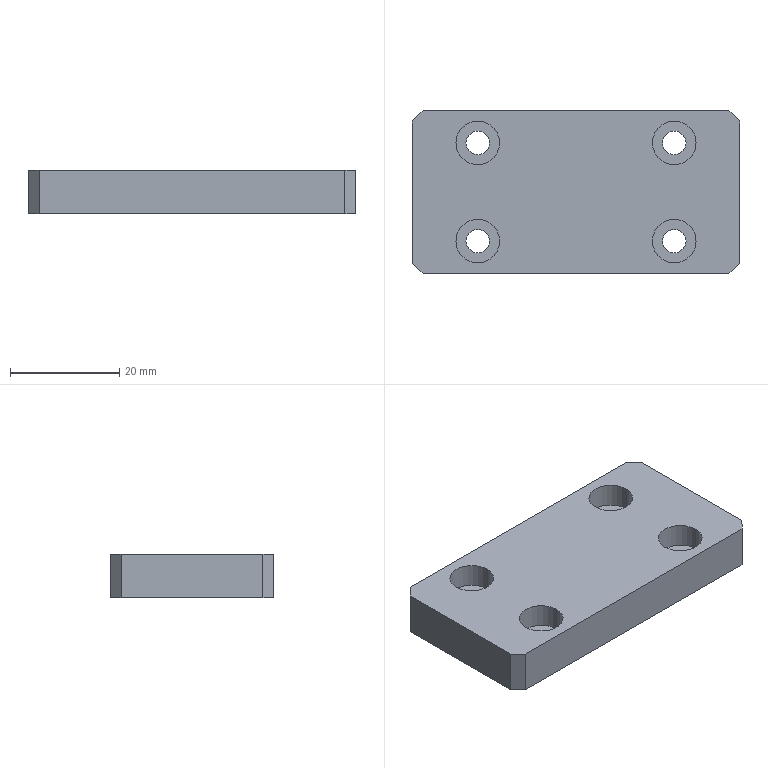Component | SolidWorks | XT-1-24-2-5 | 1 solid | 30 faces | box 60 x 30 x 8 mm | volume 13242 mm3 | cylinder 16 | plane 14 | commonest cylinder face diameters 8 x8 4.3 x8
build123d program:
from build123d import *

# Parameters (mm, degrees)
SKETCH1_W                                       = 60
SKETCH1_H                                       = 30
BOSS_EXTRUDE1_DEPTH                             = 8
M4_HEX_SOCKET_HEAD_CAP_SCREW_CBORE1_D           = 4.3
M4_HEX_SOCKET_HEAD_CAP_SCREW_CBORE1_CBORE_D     = 8
M4_HEX_SOCKET_HEAD_CAP_SCREW_CBORE1_CBORE_DEPTH = 4.4
CHAMFER1_SIZE                                   = 2


with BuildPart() as part:
    # Sketch1 → Boss-Extrude1 (new body)
    with BuildSketch(Plane.XY):
        with Locations((30, -15)):
            Rectangle(SKETCH1_W, SKETCH1_H)
    extrude(amount=BOSS_EXTRUDE1_DEPTH)

    # M4 Hex Socket Head Cap Screw CBORE1 (through all)
    with Locations(Plane.XY.offset(8)):
        with Locations((12, -6), (12, -24), (48, -6), (48, -24)):
            CounterBoreHole(M4_HEX_SOCKET_HEAD_CAP_SCREW_CBORE1_D / 2, M4_HEX_SOCKET_HEAD_CAP_SCREW_CBORE1_CBORE_D / 2, M4_HEX_SOCKET_HEAD_CAP_SCREW_CBORE1_CBORE_DEPTH)

    # Chamfer1
    chamfer1_edges = [part.edges().sort_by_distance(p)[0] for p in [
        (0, 0, 4),
        (60, 0, 4),
        (60, -30, 4),
        (0, -30, 4),
    ]]
    chamfer(chamfer1_edges, length=CHAMFER1_SIZE)


solid = part.part

# Placed as in the assembly
solid = solid.moved(Location((934.283, 92.385, -0.5), (0, 0, 0)))
STEP:
#1=CARTESIAN_POINT('',(37.098,3.401,0.122));
#2=VERTEX_POINT('',#1);
#3=CARTESIAN_POINT('',(37.413,3.401,0.122));
#4=VERTEX_POINT('',#3);
#5=CARTESIAN_POINT('',(37.255,3.401,0.122));
#6=DIRECTION('',(0.,0.,1.));
#7=DIRECTION('',(1.,0.,0.));
#8=AXIS2_PLACEMENT_3D('',#5,#6,#7);
#9=CIRCLE('',#8,0.1575);
#10=EDGE_CURVE('',#2,#4,#9,.T.);
#11=ORIENTED_EDGE('',*,*,#10,.F.);
#12=CARTESIAN_POINT('',(37.098,3.401,0.2953));
#13=VERTEX_POINT('',#12);
#14=CARTESIAN_POINT('',(37.098,3.401,0.2953));
#15=DIRECTION('',(0.,0.,1.));
#16=VECTOR('',#15,39.37);
#17=LINE('',#14,#16);
#18=EDGE_CURVE('',#2,#13,#17,.T.);
#19=ORIENTED_EDGE('',*,*,#18,.T.);
#20=CARTESIAN_POINT('',(37.413,3.401,0.2953));
#21=VERTEX_POINT('',#20);
#22=CARTESIAN_POINT('',(37.255,3.401,0.2953));
#23=DIRECTION('',(0.,0.,1.));
#24=DIRECTION('',(1.,0.,0.));
#25=AXIS2_PLACEMENT_3D('',#22,#23,#24);
#26=CIRCLE('',#25,0.1575);
#27=EDGE_CURVE('',#13,#21,#26,.T.);
#28=ORIENTED_EDGE('',*,*,#27,.T.);
#29=CARTESIAN_POINT('',(37.413,3.401,0.2953));
#30=DIRECTION('',(0.,0.,1.));
#31=VECTOR('',#30,39.37);
#32=LINE('',#29,#31);
#33=EDGE_CURVE('',#4,#21,#32,.T.);
#34=ORIENTED_EDGE('',*,*,#33,.F.);
#35=EDGE_LOOP('',(#11,#19,#28,#34));
#36=FACE_OUTER_BOUND('',#35,.T.);
#37=CARTESIAN_POINT('',(37.255,3.401,0.2953));
#38=DIRECTION('',(0.,0.,1.));
#39=DIRECTION('',(1.,0.,0.));
#40=AXIS2_PLACEMENT_3D('',#37,#38,#39);
#41=CYLINDRICAL_SURFACE('',#40,0.1575);
#42=ADVANCED_FACE('',(#36),#41,.F.);
#43=CARTESIAN_POINT('',(37.171,3.401,-0.01969));
#44=VERTEX_POINT('',#43);
#45=CARTESIAN_POINT('',(37.34,3.401,-0.01969));
#46=VERTEX_POINT('',#45);
#47=CARTESIAN_POINT('',(37.255,3.401,-0.01969));
#48=DIRECTION('',(0.,0.,1.));
#49=DIRECTION('',(1.,0.,0.));
#50=AXIS2_PLACEMENT_3D('',#47,#48,#49);
#51=CIRCLE('',#50,0.08465);
#52=EDGE_CURVE('',#44,#46,#51,.T.);
#53=ORIENTED_EDGE('',*,*,#52,.F.);
#54=CARTESIAN_POINT('',(37.171,3.401,0.122));
#55=VERTEX_POINT('',#54);
#56=CARTESIAN_POINT('',(37.171,3.401,0.2953));
#57=DIRECTION('',(0.,0.,1.));
#58=VECTOR('',#57,39.37);
#59=LINE('',#56,#58);
#60=EDGE_CURVE('',#44,#55,#59,.T.);
#61=ORIENTED_EDGE('',*,*,#60,.T.);
#62=CARTESIAN_POINT('',(37.34,3.401,0.122));
#63=VERTEX_POINT('',#62);
#64=CARTESIAN_POINT('',(37.255,3.401,0.122));
#65=DIRECTION('',(0.,0.,1.));
#66=DIRECTION('',(1.,0.,0.));
#67=AXIS2_PLACEMENT_3D('',#64,#65,#66);
#68=CIRCLE('',#67,0.08465);
#69=EDGE_CURVE('',#55,#63,#68,.T.);
#70=ORIENTED_EDGE('',*,*,#69,.T.);
#71=CARTESIAN_POINT('',(37.34,3.401,0.2953));
#72=DIRECTION('',(0.,0.,1.));
#73=VECTOR('',#72,39.37);
#74=LINE('',#71,#73);
#75=EDGE_CURVE('',#46,#63,#74,.T.);
#76=ORIENTED_EDGE('',*,*,#75,.F.);
#77=EDGE_LOOP('',(#53,#61,#70,#76));
#78=FACE_OUTER_BOUND('',#77,.T.);
#79=CARTESIAN_POINT('',(37.255,3.401,0.2953));
#80=DIRECTION('',(0.,0.,1.));
#81=DIRECTION('',(1.,0.,0.));
#82=AXIS2_PLACEMENT_3D('',#79,#80,#81);
#83=CYLINDRICAL_SURFACE('',#82,0.08465);
#84=ADVANCED_FACE('',(#78),#83,.F.);
#85=CARTESIAN_POINT('',(37.098,2.692,0.122));
#86=VERTEX_POINT('',#85);
#87=CARTESIAN_POINT('',(37.413,2.692,0.122));
#88=VERTEX_POINT('',#87);
#89=CARTESIAN_POINT('',(37.255,2.692,0.122));
#90=DIRECTION('',(0.,0.,1.));
#91=DIRECTION('',(1.,0.,0.));
#92=AXIS2_PLACEMENT_3D('',#89,#90,#91);
#93=CIRCLE('',#92,0.1575);
#94=EDGE_CURVE('',#86,#88,#93,.T.);
#95=ORIENTED_EDGE('',*,*,#94,.F.);
#96=CARTESIAN_POINT('',(37.098,2.692,0.2953));
#97=VERTEX_POINT('',#96);
#98=CARTESIAN_POINT('',(37.098,2.692,0.2953));
#99=DIRECTION('',(0.,0.,1.));
#100=VECTOR('',#99,39.37);
#101=LINE('',#98,#100);
#102=EDGE_CURVE('',#86,#97,#101,.T.);
#103=ORIENTED_EDGE('',*,*,#102,.T.);
#104=CARTESIAN_POINT('',(37.413,2.692,0.2953));
#105=VERTEX_POINT('',#104);
#106=CARTESIAN_POINT('',(37.255,2.692,0.2953));
#107=DIRECTION('',(0.,0.,1.));
#108=DIRECTION('',(1.,0.,0.));
#109=AXIS2_PLACEMENT_3D('',#106,#107,#108);
#110=CIRCLE('',#109,0.1575);
#111=EDGE_CURVE('',#97,#105,#110,.T.);
#112=ORIENTED_EDGE('',*,*,#111,.T.);
#113=CARTESIAN_POINT('',(37.413,2.692,0.2953));
#114=DIRECTION('',(0.,0.,1.));
#115=VECTOR('',#114,39.37);
#116=LINE('',#113,#115);
#117=EDGE_CURVE('',#88,#105,#116,.T.);
#118=ORIENTED_EDGE('',*,*,#117,.F.);
#119=EDGE_LOOP('',(#95,#103,#112,#118));
#120=FACE_OUTER_BOUND('',#119,.T.);
#121=CARTESIAN_POINT('',(37.255,2.692,0.2953));
#122=DIRECTION('',(0.,0.,1.));
#123=DIRECTION('',(1.,0.,0.));
#124=AXIS2_PLACEMENT_3D('',#121,#122,#123);
#125=CYLINDRICAL_SURFACE('',#124,0.1575);
#126=ADVANCED_FACE('',(#120),#125,.F.);
#127=CARTESIAN_POINT('',(37.171,2.692,-0.01969));
#128=VERTEX_POINT('',#127);
#129=CARTESIAN_POINT('',(37.34,2.692,-0.01969));
#130=VERTEX_POINT('',#129);
#131=CARTESIAN_POINT('',(37.255,2.692,-0.01969));
#132=DIRECTION('',(0.,0.,1.));
#133=DIRECTION('',(1.,0.,0.));
#134=AXIS2_PLACEMENT_3D('',#131,#132,#133);
#135=CIRCLE('',#134,0.08465);
#136=EDGE_CURVE('',#128,#130,#135,.T.);
#137=ORIENTED_EDGE('',*,*,#136,.F.);
#138=CARTESIAN_POINT('',(37.171,2.692,0.122));
#139=VERTEX_POINT('',#138);
#140=CARTESIAN_POINT('',(37.171,2.692,0.2953));
#141=DIRECTION('',(0.,0.,1.));
#142=VECTOR('',#141,39.37);
#143=LINE('',#140,#142);
#144=EDGE_CURVE('',#128,#139,#143,.T.);
#145=ORIENTED_EDGE('',*,*,#144,.T.);
#146=CARTESIAN_POINT('',(37.34,2.692,0.122));
#147=VERTEX_POINT('',#146);
#148=CARTESIAN_POINT('',(37.255,2.692,0.122));
#149=DIRECTION('',(0.,0.,1.));
#150=DIRECTION('',(1.,0.,0.));
#151=AXIS2_PLACEMENT_3D('',#148,#149,#150);
#152=CIRCLE('',#151,0.08465);
#153=EDGE_CURVE('',#139,#147,#152,.T.);
#154=ORIENTED_EDGE('',*,*,#153,.T.);
#155=CARTESIAN_POINT('',(37.34,2.692,0.2953));
#156=DIRECTION('',(0.,0.,1.));
#157=VECTOR('',#156,39.37);
#158=LINE('',#155,#157);
#159=EDGE_CURVE('',#130,#147,#158,.T.);
#160=ORIENTED_EDGE('',*,*,#159,.F.);
#161=EDGE_LOOP('',(#137,#145,#154,#160));
#162=FACE_OUTER_BOUND('',#161,.T.);
#163=CARTESIAN_POINT('',(37.255,2.692,0.2953));
#164=DIRECTION('',(0.,0.,1.));
#165=DIRECTION('',(1.,0.,0.));
#166=AXIS2_PLACEMENT_3D('',#163,#164,#165);
#167=CYLINDRICAL_SURFACE('',#166,0.08465);
#168=ADVANCED_FACE('',(#162),#167,.F.);
#169=CARTESIAN_POINT('',(38.515,3.401,0.122));
#170=VERTEX_POINT('',#169);
#171=CARTESIAN_POINT('',(38.83,3.401,0.122));
#172=VERTEX_POINT('',#171);
#173=CARTESIAN_POINT('',(38.673,3.401,0.122));
#174=DIRECTION('',(0.,0.,1.));
#175=DIRECTION('',(1.,0.,0.));
#176=AXIS2_PLACEMENT_3D('',#173,#174,#175);
#177=CIRCLE('',#176,0.1575);
#178=EDGE_CURVE('',#170,#172,#177,.T.);
#179=ORIENTED_EDGE('',*,*,#178,.F.);
#180=CARTESIAN_POINT('',(38.515,3.401,0.2953));
#181=VERTEX_POINT('',#180);
#182=CARTESIAN_POINT('',(38.515,3.401,0.2953));
#183=DIRECTION('',(0.,0.,1.));
#184=VECTOR('',#183,39.37);
#185=LINE('',#182,#184);
#186=EDGE_CURVE('',#170,#181,#185,.T.);
#187=ORIENTED_EDGE('',*,*,#186,.T.);
#188=CARTESIAN_POINT('',(38.83,3.401,0.2953));
#189=VERTEX_POINT('',#188);
#190=CARTESIAN_POINT('',(38.673,3.401,0.2953));
#191=DIRECTION('',(0.,0.,1.));
#192=DIRECTION('',(1.,0.,0.));
#193=AXIS2_PLACEMENT_3D('',#190,#191,#192);
#194=CIRCLE('',#193,0.1575);
#195=EDGE_CURVE('',#181,#189,#194,.T.);
#196=ORIENTED_EDGE('',*,*,#195,.T.);
#197=CARTESIAN_POINT('',(38.83,3.401,0.2953));
#198=DIRECTION('',(0.,0.,1.));
#199=VECTOR('',#198,39.37);
#200=LINE('',#197,#199);
#201=EDGE_CURVE('',#172,#189,#200,.T.);
#202=ORIENTED_EDGE('',*,*,#201,.F.);
#203=EDGE_LOOP('',(#179,#187,#196,#202));
#204=FACE_OUTER_BOUND('',#203,.T.);
#205=CARTESIAN_POINT('',(38.673,3.401,0.2953));
#206=DIRECTION('',(0.,0.,1.));
#207=DIRECTION('',(1.,0.,0.));
#208=AXIS2_PLACEMENT_3D('',#205,#206,#207);
#209=CYLINDRICAL_SURFACE('',#208,0.1575);
#210=ADVANCED_FACE('',(#204),#209,.F.);
#211=CARTESIAN_POINT('',(38.588,3.401,-0.01969));
#212=VERTEX_POINT('',#211);
#213=CARTESIAN_POINT('',(38.757,3.401,-0.01969));
#214=VERTEX_POINT('',#213);
#215=CARTESIAN_POINT('',(38.673,3.401,-0.01969));
#216=DIRECTION('',(0.,0.,1.));
#217=DIRECTION('',(1.,0.,0.));
#218=AXIS2_PLACEMENT_3D('',#215,#216,#217);
#219=CIRCLE('',#218,0.08465);
#220=EDGE_CURVE('',#212,#214,#219,.T.);
#221=ORIENTED_EDGE('',*,*,#220,.F.);
#222=CARTESIAN_POINT('',(38.588,3.401,0.122));
#223=VERTEX_POINT('',#222);
#224=CARTESIAN_POINT('',(38.588,3.401,0.2953));
#225=DIRECTION('',(0.,0.,1.));
#226=VECTOR('',#225,39.37);
#227=LINE('',#224,#226);
#228=EDGE_CURVE('',#212,#223,#227,.T.);
#229=ORIENTED_EDGE('',*,*,#228,.T.);
#230=CARTESIAN_POINT('',(38.757,3.401,0.122));
#231=VERTEX_POINT('',#230);
#232=CARTESIAN_POINT('',(38.673,3.401,0.122));
#233=DIRECTION('',(0.,0.,1.));
#234=DIRECTION('',(1.,0.,0.));
#235=AXIS2_PLACEMENT_3D('',#232,#233,#234);
#236=CIRCLE('',#235,0.08465);
#237=EDGE_CURVE('',#223,#231,#236,.T.);
#238=ORIENTED_EDGE('',*,*,#237,.T.);
#239=CARTESIAN_POINT('',(38.757,3.401,0.2953));
#240=DIRECTION('',(0.,0.,1.));
#241=VECTOR('',#240,39.37);
#242=LINE('',#239,#241);
#243=EDGE_CURVE('',#214,#231,#242,.T.);
#244=ORIENTED_EDGE('',*,*,#243,.F.);
#245=EDGE_LOOP('',(#221,#229,#238,#244));
#246=FACE_OUTER_BOUND('',#245,.T.);
#247=CARTESIAN_POINT('',(38.673,3.401,0.2953));
#248=DIRECTION('',(0.,0.,1.));
#249=DIRECTION('',(1.,0.,0.));
#250=AXIS2_PLACEMENT_3D('',#247,#248,#249);
#251=CYLINDRICAL_SURFACE('',#250,0.08465);
#252=ADVANCED_FACE('',(#246),#251,.F.);
#253=CARTESIAN_POINT('',(38.515,2.692,0.122));
#254=VERTEX_POINT('',#253);
#255=CARTESIAN_POINT('',(38.83,2.692,0.122));
#256=VERTEX_POINT('',#255);
#257=CARTESIAN_POINT('',(38.673,2.692,0.122));
#258=DIRECTION('',(0.,0.,1.));
#259=DIRECTION('',(1.,0.,0.));
#260=AXIS2_PLACEMENT_3D('',#257,#258,#259);
#261=CIRCLE('',#260,0.1575);
#262=EDGE_CURVE('',#254,#256,#261,.T.);
#263=ORIENTED_EDGE('',*,*,#262,.F.);
#264=CARTESIAN_POINT('',(38.515,2.692,0.2953));
#265=VERTEX_POINT('',#264);
#266=CARTESIAN_POINT('',(38.515,2.692,0.2953));
#267=DIRECTION('',(0.,0.,1.));
#268=VECTOR('',#267,39.37);
#269=LINE('',#266,#268);
#270=EDGE_CURVE('',#254,#265,#269,.T.);
#271=ORIENTED_EDGE('',*,*,#270,.T.);
#272=CARTESIAN_POINT('',(38.83,2.692,0.2953));
#273=VERTEX_POINT('',#272);
#274=CARTESIAN_POINT('',(38.673,2.692,0.2953));
#275=DIRECTION('',(0.,0.,1.));
#276=DIRECTION('',(1.,0.,0.));
#277=AXIS2_PLACEMENT_3D('',#274,#275,#276);
#278=CIRCLE('',#277,0.1575);
#279=EDGE_CURVE('',#265,#273,#278,.T.);
#280=ORIENTED_EDGE('',*,*,#279,.T.);
#281=CARTESIAN_POINT('',(38.83,2.692,0.2953));
#282=DIRECTION('',(0.,0.,1.));
#283=VECTOR('',#282,39.37);
#284=LINE('',#281,#283);
#285=EDGE_CURVE('',#256,#273,#284,.T.);
#286=ORIENTED_EDGE('',*,*,#285,.F.);
#287=EDGE_LOOP('',(#263,#271,#280,#286));
#288=FACE_OUTER_BOUND('',#287,.T.);
#289=CARTESIAN_POINT('',(38.673,2.692,0.2953));
#290=DIRECTION('',(0.,0.,1.));
#291=DIRECTION('',(1.,0.,0.));
#292=AXIS2_PLACEMENT_3D('',#289,#290,#291);
#293=CYLINDRICAL_SURFACE('',#292,0.1575);
#294=ADVANCED_FACE('',(#288),#293,.F.);
#295=CARTESIAN_POINT('',(38.588,2.692,-0.01969));
#296=VERTEX_POINT('',#295);
#297=CARTESIAN_POINT('',(38.757,2.692,-0.01969));
#298=VERTEX_POINT('',#297);
#299=CARTESIAN_POINT('',(38.673,2.692,-0.01969));
#300=DIRECTION('',(0.,0.,1.));
#301=DIRECTION('',(1.,0.,0.));
#302=AXIS2_PLACEMENT_3D('',#299,#300,#301);
#303=CIRCLE('',#302,0.08465);
#304=EDGE_CURVE('',#296,#298,#303,.T.);
#305=ORIENTED_EDGE('',*,*,#304,.F.);
#306=CARTESIAN_POINT('',(38.588,2.692,0.122));
#307=VERTEX_POINT('',#306);
#308=CARTESIAN_POINT('',(38.588,2.692,0.2953));
#309=DIRECTION('',(0.,0.,1.));
#310=VECTOR('',#309,39.37);
#311=LINE('',#308,#310);
#312=EDGE_CURVE('',#296,#307,#311,.T.);
#313=ORIENTED_EDGE('',*,*,#312,.T.);
#314=CARTESIAN_POINT('',(38.757,2.692,0.122));
#315=VERTEX_POINT('',#314);
#316=CARTESIAN_POINT('',(38.673,2.692,0.122));
#317=DIRECTION('',(0.,0.,1.));
#318=DIRECTION('',(1.,0.,0.));
#319=AXIS2_PLACEMENT_3D('',#316,#317,#318);
#320=CIRCLE('',#319,0.08465);
#321=EDGE_CURVE('',#307,#315,#320,.T.);
#322=ORIENTED_EDGE('',*,*,#321,.T.);
#323=CARTESIAN_POINT('',(38.757,2.692,0.2953));
#324=DIRECTION('',(0.,0.,1.));
#325=VECTOR('',#324,39.37);
#326=LINE('',#323,#325);
#327=EDGE_CURVE('',#298,#315,#326,.T.);
#328=ORIENTED_EDGE('',*,*,#327,.F.);
#329=EDGE_LOOP('',(#305,#313,#322,#328));
#330=FACE_OUTER_BOUND('',#329,.T.);
#331=CARTESIAN_POINT('',(38.673,2.692,0.2953));
#332=DIRECTION('',(0.,0.,1.));
#333=DIRECTION('',(1.,0.,0.));
#334=AXIS2_PLACEMENT_3D('',#331,#332,#333);
#335=CYLINDRICAL_SURFACE('',#334,0.08465);
#336=ADVANCED_FACE('',(#330),#335,.F.);
#337=CARTESIAN_POINT('',(36.783,3.558,-0.01969));
#338=VERTEX_POINT('',#337);
#339=CARTESIAN_POINT('',(36.783,2.535,-0.01969));
#340=VERTEX_POINT('',#339);
#341=CARTESIAN_POINT('',(36.783,3.637,-0.01969));
#342=DIRECTION('',(0.,-1.,0.));
#343=VECTOR('',#342,39.37);
#344=LINE('',#341,#343);
#345=EDGE_CURVE('',#338,#340,#344,.T.);
#346=ORIENTED_EDGE('',*,*,#345,.T.);
#347=CARTESIAN_POINT('',(36.783,2.535,0.2953));
#348=VERTEX_POINT('',#347);
#349=CARTESIAN_POINT('',(36.783,2.535,0.2953));
#350=DIRECTION('',(0.,0.,1.));
#351=VECTOR('',#350,39.37);
#352=LINE('',#349,#351);
#353=EDGE_CURVE('',#340,#348,#352,.T.);
#354=ORIENTED_EDGE('',*,*,#353,.T.);
#355=CARTESIAN_POINT('',(36.783,3.558,0.2953));
#356=VERTEX_POINT('',#355);
#357=CARTESIAN_POINT('',(36.783,3.637,0.2953));
#358=DIRECTION('',(0.,-1.,0.));
#359=VECTOR('',#358,39.37);
#360=LINE('',#357,#359);
#361=EDGE_CURVE('',#356,#348,#360,.T.);
#362=ORIENTED_EDGE('',*,*,#361,.F.);
#363=CARTESIAN_POINT('',(36.783,3.558,0.2953));
#364=DIRECTION('',(0.,0.,-1.));
#365=VECTOR('',#364,39.37);
#366=LINE('',#363,#365);
#367=EDGE_CURVE('',#356,#338,#366,.T.);
#368=ORIENTED_EDGE('',*,*,#367,.T.);
#369=EDGE_LOOP('',(#346,#354,#362,#368));
#370=FACE_OUTER_BOUND('',#369,.T.);
#371=CARTESIAN_POINT('',(36.783,3.637,0.2953));
#372=DIRECTION('',(1.,0.,0.));
#373=DIRECTION('',(-0.,1.,0.));
#374=AXIS2_PLACEMENT_3D('',#371,#372,#373);
#375=PLANE('',#374);
#376=ADVANCED_FACE('',(#370),#375,.F.);
#377=CARTESIAN_POINT('',(36.862,2.456,-0.01969));
#378=VERTEX_POINT('',#377);
#379=CARTESIAN_POINT('',(39.066,2.456,-0.01969));
#380=VERTEX_POINT('',#379);
#381=CARTESIAN_POINT('',(36.783,2.456,-0.01969));
#382=DIRECTION('',(1.,0.,0.));
#383=VECTOR('',#382,39.37);
#384=LINE('',#381,#383);
#385=EDGE_CURVE('',#378,#380,#384,.T.);
#386=ORIENTED_EDGE('',*,*,#385,.T.);
#387=CARTESIAN_POINT('',(39.066,2.456,0.2953));
#388=VERTEX_POINT('',#387);
#389=CARTESIAN_POINT('',(39.066,2.456,0.2953));
#390=DIRECTION('',(0.,0.,1.));
#391=VECTOR('',#390,39.37);
#392=LINE('',#389,#391);
#393=EDGE_CURVE('',#380,#388,#392,.T.);
#394=ORIENTED_EDGE('',*,*,#393,.T.);
#395=CARTESIAN_POINT('',(36.862,2.456,0.2953));
#396=VERTEX_POINT('',#395);
#397=CARTESIAN_POINT('',(36.783,2.456,0.2953));
#398=DIRECTION('',(1.,0.,0.));
#399=VECTOR('',#398,39.37);
#400=LINE('',#397,#399);
#401=EDGE_CURVE('',#396,#388,#400,.T.);
#402=ORIENTED_EDGE('',*,*,#401,.F.);
#403=CARTESIAN_POINT('',(36.862,2.456,0.2953));
#404=DIRECTION('',(0.,0.,-1.));
#405=VECTOR('',#404,39.37);
#406=LINE('',#403,#405);
#407=EDGE_CURVE('',#396,#378,#406,.T.);
#408=ORIENTED_EDGE('',*,*,#407,.T.);
#409=EDGE_LOOP('',(#386,#394,#402,#408));
#410=FACE_OUTER_BOUND('',#409,.T.);
#411=CARTESIAN_POINT('',(36.783,2.456,0.2953));
#412=DIRECTION('',(0.,1.,0.));
#413=DIRECTION('',(0.,0.,1.));
#414=AXIS2_PLACEMENT_3D('',#411,#412,#413);
#415=PLANE('',#414);
#416=ADVANCED_FACE('',(#410),#415,.F.);
#417=CARTESIAN_POINT('',(39.145,2.535,-0.01969));
#418=VERTEX_POINT('',#417);
#419=CARTESIAN_POINT('',(39.145,3.558,-0.01969));
#420=VERTEX_POINT('',#419);
#421=CARTESIAN_POINT('',(39.145,3.637,-0.01969));
#422=DIRECTION('',(-0.,1.,0.));
#423=VECTOR('',#422,39.37);
#424=LINE('',#421,#423);
#425=EDGE_CURVE('',#418,#420,#424,.T.);
#426=ORIENTED_EDGE('',*,*,#425,.T.);
#427=CARTESIAN_POINT('',(39.145,3.558,0.2953));
#428=VERTEX_POINT('',#427);
#429=CARTESIAN_POINT('',(39.145,3.558,0.2953));
#430=DIRECTION('',(0.,0.,1.));
#431=VECTOR('',#430,39.37);
#432=LINE('',#429,#431);
#433=EDGE_CURVE('',#420,#428,#432,.T.);
#434=ORIENTED_EDGE('',*,*,#433,.T.);
#435=CARTESIAN_POINT('',(39.145,2.535,0.2953));
#436=VERTEX_POINT('',#435);
#437=CARTESIAN_POINT('',(39.145,3.637,0.2953));
#438=DIRECTION('',(-0.,1.,0.));
#439=VECTOR('',#438,39.37);
#440=LINE('',#437,#439);
#441=EDGE_CURVE('',#436,#428,#440,.T.);
#442=ORIENTED_EDGE('',*,*,#441,.F.);
#443=CARTESIAN_POINT('',(39.145,2.535,0.2953));
#444=DIRECTION('',(0.,0.,-1.));
#445=VECTOR('',#444,39.37);
#446=LINE('',#443,#445);
#447=EDGE_CURVE('',#436,#418,#446,.T.);
#448=ORIENTED_EDGE('',*,*,#447,.T.);
#449=EDGE_LOOP('',(#426,#434,#442,#448));
#450=FACE_OUTER_BOUND('',#449,.T.);
#451=CARTESIAN_POINT('',(39.145,3.637,0.2953));
#452=DIRECTION('',(-1.,-0.,0.));
#453=DIRECTION('',(0.,-1.,0.));
#454=AXIS2_PLACEMENT_3D('',#451,#452,#453);
#455=PLANE('',#454);
#456=ADVANCED_FACE('',(#450),#455,.F.);
#457=CARTESIAN_POINT('',(39.066,3.637,0.2953));
#458=VERTEX_POINT('',#457);
#459=CARTESIAN_POINT('',(36.862,3.637,0.2953));
#460=VERTEX_POINT('',#459);
#461=CARTESIAN_POINT('',(36.783,3.637,0.2953));
#462=DIRECTION('',(-1.,0.,0.));
#463=VECTOR('',#462,39.37);
#464=LINE('',#461,#463);
#465=EDGE_CURVE('',#458,#460,#464,.T.);
#466=ORIENTED_EDGE('',*,*,#465,.F.);
#467=CARTESIAN_POINT('',(39.066,3.637,-0.01969));
#468=VERTEX_POINT('',#467);
#469=CARTESIAN_POINT('',(39.066,3.637,0.2953));
#470=DIRECTION('',(0.,0.,-1.));
#471=VECTOR('',#470,39.37);
#472=LINE('',#469,#471);
#473=EDGE_CURVE('',#458,#468,#472,.T.);
#474=ORIENTED_EDGE('',*,*,#473,.T.);
#475=CARTESIAN_POINT('',(36.862,3.637,-0.01969));
#476=VERTEX_POINT('',#475);
#477=CARTESIAN_POINT('',(36.783,3.637,-0.01969));
#478=DIRECTION('',(-1.,0.,0.));
#479=VECTOR('',#478,39.37);
#480=LINE('',#477,#479);
#481=EDGE_CURVE('',#468,#476,#480,.T.);
#482=ORIENTED_EDGE('',*,*,#481,.T.);
#483=CARTESIAN_POINT('',(36.862,3.637,0.2953));
#484=DIRECTION('',(0.,0.,1.));
#485=VECTOR('',#484,39.37);
#486=LINE('',#483,#485);
#487=EDGE_CURVE('',#476,#460,#486,.T.);
#488=ORIENTED_EDGE('',*,*,#487,.T.);
#489=EDGE_LOOP('',(#466,#474,#482,#488));
#490=FACE_OUTER_BOUND('',#489,.T.);
#491=CARTESIAN_POINT('',(36.783,3.637,0.2953));
#492=DIRECTION('',(0.,-1.,0.));
#493=DIRECTION('',(0.,0.,-1.));
#494=AXIS2_PLACEMENT_3D('',#491,#492,#493);
#495=PLANE('',#494);
#496=ADVANCED_FACE('',(#490),#495,.F.);
#497=CARTESIAN_POINT('',(37.255,3.401,0.2953));
#498=DIRECTION('',(0.,0.,1.));
#499=DIRECTION('',(1.,0.,0.));
#500=AXIS2_PLACEMENT_3D('',#497,#498,#499);
#501=CIRCLE('',#500,0.1575);
#502=EDGE_CURVE('',#21,#13,#501,.T.);
#503=ORIENTED_EDGE('',*,*,#502,.F.);
#504=ORIENTED_EDGE('',*,*,#27,.F.);
#505=EDGE_LOOP('',(#503,#504));
#506=FACE_BOUND('',#505,.T.);
#507=CARTESIAN_POINT('',(37.255,2.692,0.2953));
#508=DIRECTION('',(0.,0.,1.));
#509=DIRECTION('',(1.,0.,0.));
#510=AXIS2_PLACEMENT_3D('',#507,#508,#509);
#511=CIRCLE('',#510,0.1575);
#512=EDGE_CURVE('',#105,#97,#511,.T.);
#513=ORIENTED_EDGE('',*,*,#512,.F.);
#514=ORIENTED_EDGE('',*,*,#111,.F.);
#515=EDGE_LOOP('',(#513,#514));
#516=FACE_BOUND('',#515,.T.);
#517=CARTESIAN_POINT('',(38.673,3.401,0.2953));
#518=DIRECTION('',(0.,0.,1.));
#519=DIRECTION('',(1.,0.,0.));
#520=AXIS2_PLACEMENT_3D('',#517,#518,#519);
#521=CIRCLE('',#520,0.1575);
#522=EDGE_CURVE('',#189,#181,#521,.T.);
#523=ORIENTED_EDGE('',*,*,#522,.F.);
#524=ORIENTED_EDGE('',*,*,#195,.F.);
#525=EDGE_LOOP('',(#523,#524));
#526=FACE_BOUND('',#525,.T.);
#527=CARTESIAN_POINT('',(38.673,2.692,0.2953));
#528=DIRECTION('',(0.,0.,1.));
#529=DIRECTION('',(1.,0.,0.));
#530=AXIS2_PLACEMENT_3D('',#527,#528,#529);
#531=CIRCLE('',#530,0.1575);
#532=EDGE_CURVE('',#273,#265,#531,.T.);
#533=ORIENTED_EDGE('',*,*,#532,.F.);
#534=ORIENTED_EDGE('',*,*,#279,.F.);
#535=EDGE_LOOP('',(#533,#534));
#536=FACE_BOUND('',#535,.T.);
#537=ORIENTED_EDGE('',*,*,#441,.T.);
#538=CARTESIAN_POINT('',(38.515,4.188,0.2953));
#539=DIRECTION('',(-0.7071,0.7071,0.));
#540=VECTOR('',#539,39.37);
#541=LINE('',#538,#540);
#542=EDGE_CURVE('',#428,#458,#541,.T.);
#543=ORIENTED_EDGE('',*,*,#542,.T.);
#544=ORIENTED_EDGE('',*,*,#465,.T.);
#545=CARTESIAN_POINT('',(36.232,3.007,0.2953));
#546=DIRECTION('',(-0.7071,-0.7071,0.));
#547=VECTOR('',#546,39.37);
#548=LINE('',#545,#547);
#549=EDGE_CURVE('',#460,#356,#548,.T.);
#550=ORIENTED_EDGE('',*,*,#549,.T.);
#551=ORIENTED_EDGE('',*,*,#361,.T.);
#552=CARTESIAN_POINT('',(36.822,2.495,0.2953));
#553=DIRECTION('',(0.7071,-0.7071,0.));
#554=VECTOR('',#553,39.37);
#555=LINE('',#552,#554);
#556=EDGE_CURVE('',#348,#396,#555,.T.);
#557=ORIENTED_EDGE('',*,*,#556,.T.);
#558=ORIENTED_EDGE('',*,*,#401,.T.);
#559=CARTESIAN_POINT('',(37.925,1.314,0.2953));
#560=DIRECTION('',(0.7071,0.7071,0.));
#561=VECTOR('',#560,39.37);
#562=LINE('',#559,#561);
#563=EDGE_CURVE('',#388,#436,#562,.T.);
#564=ORIENTED_EDGE('',*,*,#563,.T.);
#565=EDGE_LOOP('',(#537,#543,#544,#550,#551,#557,#558,#564));
#566=FACE_OUTER_BOUND('',#565,.T.);
#567=CARTESIAN_POINT('',(36.783,2.456,0.2953));
#568=DIRECTION('',(0.,0.,1.));
#569=DIRECTION('',(1.,0.,0.));
#570=AXIS2_PLACEMENT_3D('',#567,#568,#569);
#571=PLANE('',#570);
#572=ADVANCED_FACE('',(#506,#516,#526,#536,#566),#571,.T.);
#573=CARTESIAN_POINT('',(37.255,3.401,-0.01969));
#574=DIRECTION('',(0.,0.,1.));
#575=DIRECTION('',(1.,0.,0.));
#576=AXIS2_PLACEMENT_3D('',#573,#574,#575);
#577=CIRCLE('',#576,0.08465);
#578=EDGE_CURVE('',#46,#44,#577,.T.);
#579=ORIENTED_EDGE('',*,*,#578,.T.);
#580=ORIENTED_EDGE('',*,*,#52,.T.);
#581=EDGE_LOOP('',(#579,#580));
#582=FACE_BOUND('',#581,.T.);
#583=CARTESIAN_POINT('',(37.255,2.692,-0.01969));
#584=DIRECTION('',(0.,0.,1.));
#585=DIRECTION('',(1.,0.,0.));
#586=AXIS2_PLACEMENT_3D('',#583,#584,#585);
#587=CIRCLE('',#586,0.08465);
#588=EDGE_CURVE('',#130,#128,#587,.T.);
#589=ORIENTED_EDGE('',*,*,#588,.T.);
#590=ORIENTED_EDGE('',*,*,#136,.T.);
#591=EDGE_LOOP('',(#589,#590));
#592=FACE_BOUND('',#591,.T.);
#593=CARTESIAN_POINT('',(38.673,3.401,-0.01969));
#594=DIRECTION('',(0.,0.,1.));
#595=DIRECTION('',(1.,0.,0.));
#596=AXIS2_PLACEMENT_3D('',#593,#594,#595);
#597=CIRCLE('',#596,0.08465);
#598=EDGE_CURVE('',#214,#212,#597,.T.);
#599=ORIENTED_EDGE('',*,*,#598,.T.);
#600=ORIENTED_EDGE('',*,*,#220,.T.);
#601=EDGE_LOOP('',(#599,#600));
#602=FACE_BOUND('',#601,.T.);
#603=CARTESIAN_POINT('',(38.673,2.692,-0.01969));
#604=DIRECTION('',(0.,0.,1.));
#605=DIRECTION('',(1.,0.,0.));
#606=AXIS2_PLACEMENT_3D('',#603,#604,#605);
#607=CIRCLE('',#606,0.08465);
#608=EDGE_CURVE('',#298,#296,#607,.T.);
#609=ORIENTED_EDGE('',*,*,#608,.T.);
#610=ORIENTED_EDGE('',*,*,#304,.T.);
#611=EDGE_LOOP('',(#609,#610));
#612=FACE_BOUND('',#611,.T.);
#613=ORIENTED_EDGE('',*,*,#481,.F.);
#614=CARTESIAN_POINT('',(39.066,3.637,-0.01969));
#615=DIRECTION('',(0.7071,-0.7071,0.));
#616=VECTOR('',#615,39.37);
#617=LINE('',#614,#616);
#618=EDGE_CURVE('',#468,#420,#617,.T.);
#619=ORIENTED_EDGE('',*,*,#618,.T.);
#620=ORIENTED_EDGE('',*,*,#425,.F.);
#621=CARTESIAN_POINT('',(39.145,2.535,-0.01969));
#622=DIRECTION('',(-0.7071,-0.7071,0.));
#623=VECTOR('',#622,39.37);
#624=LINE('',#621,#623);
#625=EDGE_CURVE('',#418,#380,#624,.T.);
#626=ORIENTED_EDGE('',*,*,#625,.T.);
#627=ORIENTED_EDGE('',*,*,#385,.F.);
#628=CARTESIAN_POINT('',(36.862,2.456,-0.01969));
#629=DIRECTION('',(-0.7071,0.7071,0.));
#630=VECTOR('',#629,39.37);
#631=LINE('',#628,#630);
#632=EDGE_CURVE('',#378,#340,#631,.T.);
#633=ORIENTED_EDGE('',*,*,#632,.T.);
#634=ORIENTED_EDGE('',*,*,#345,.F.);
#635=CARTESIAN_POINT('',(36.783,3.558,-0.01969));
#636=DIRECTION('',(0.7071,0.7071,0.));
#637=VECTOR('',#636,39.37);
#638=LINE('',#635,#637);
#639=EDGE_CURVE('',#338,#476,#638,.T.);
#640=ORIENTED_EDGE('',*,*,#639,.T.);
#641=EDGE_LOOP('',(#613,#619,#620,#626,#627,#633,#634,#640));
#642=FACE_OUTER_BOUND('',#641,.T.);
#643=CARTESIAN_POINT('',(36.783,2.456,-0.01969));
#644=DIRECTION('',(0.,0.,1.));
#645=DIRECTION('',(1.,0.,0.));
#646=AXIS2_PLACEMENT_3D('',#643,#644,#645);
#647=PLANE('',#646);
#648=ADVANCED_FACE('',(#582,#592,#602,#612,#642),#647,.F.);
#649=ORIENTED_EDGE('',*,*,#312,.F.);
#650=ORIENTED_EDGE('',*,*,#608,.F.);
#651=ORIENTED_EDGE('',*,*,#327,.T.);
#652=CARTESIAN_POINT('',(38.673,2.692,0.122));
#653=DIRECTION('',(0.,0.,1.));
#654=DIRECTION('',(1.,0.,0.));
#655=AXIS2_PLACEMENT_3D('',#652,#653,#654);
#656=CIRCLE('',#655,0.08465);
#657=EDGE_CURVE('',#315,#307,#656,.T.);
#658=ORIENTED_EDGE('',*,*,#657,.T.);
#659=EDGE_LOOP('',(#649,#650,#651,#658));
#660=FACE_OUTER_BOUND('',#659,.T.);
#661=CARTESIAN_POINT('',(38.673,2.692,0.2953));
#662=DIRECTION('',(0.,0.,1.));
#663=DIRECTION('',(1.,0.,0.));
#664=AXIS2_PLACEMENT_3D('',#661,#662,#663);
#665=CYLINDRICAL_SURFACE('',#664,0.08465);
#666=ADVANCED_FACE('',(#660),#665,.F.);
#667=ORIENTED_EDGE('',*,*,#657,.F.);
#668=ORIENTED_EDGE('',*,*,#321,.F.);
#669=EDGE_LOOP('',(#667,#668));
#670=FACE_BOUND('',#669,.T.);
#671=CARTESIAN_POINT('',(38.673,2.692,0.122));
#672=DIRECTION('',(0.,0.,1.));
#673=DIRECTION('',(1.,0.,0.));
#674=AXIS2_PLACEMENT_3D('',#671,#672,#673);
#675=CIRCLE('',#674,0.1575);
#676=EDGE_CURVE('',#256,#254,#675,.T.);
#677=ORIENTED_EDGE('',*,*,#676,.T.);
#678=ORIENTED_EDGE('',*,*,#262,.T.);
#679=EDGE_LOOP('',(#677,#678));
#680=FACE_OUTER_BOUND('',#679,.T.);
#681=CARTESIAN_POINT('',(38.757,2.692,0.122));
#682=DIRECTION('',(0.,0.,-1.));
#683=DIRECTION('',(-1.,0.,0.));
#684=AXIS2_PLACEMENT_3D('',#681,#682,#683);
#685=PLANE('',#684);
#686=ADVANCED_FACE('',(#670,#680),#685,.F.);
#687=ORIENTED_EDGE('',*,*,#270,.F.);
#688=ORIENTED_EDGE('',*,*,#676,.F.);
#689=ORIENTED_EDGE('',*,*,#285,.T.);
#690=ORIENTED_EDGE('',*,*,#532,.T.);
#691=EDGE_LOOP('',(#687,#688,#689,#690));
#692=FACE_OUTER_BOUND('',#691,.T.);
#693=CARTESIAN_POINT('',(38.673,2.692,0.2953));
#694=DIRECTION('',(0.,0.,1.));
#695=DIRECTION('',(1.,0.,0.));
#696=AXIS2_PLACEMENT_3D('',#693,#694,#695);
#697=CYLINDRICAL_SURFACE('',#696,0.1575);
#698=ADVANCED_FACE('',(#692),#697,.F.);
#699=ORIENTED_EDGE('',*,*,#228,.F.);
#700=ORIENTED_EDGE('',*,*,#598,.F.);
#701=ORIENTED_EDGE('',*,*,#243,.T.);
#702=CARTESIAN_POINT('',(38.673,3.401,0.122));
#703=DIRECTION('',(0.,0.,1.));
#704=DIRECTION('',(1.,0.,0.));
#705=AXIS2_PLACEMENT_3D('',#702,#703,#704);
#706=CIRCLE('',#705,0.08465);
#707=EDGE_CURVE('',#231,#223,#706,.T.);
#708=ORIENTED_EDGE('',*,*,#707,.T.);
#709=EDGE_LOOP('',(#699,#700,#701,#708));
#710=FACE_OUTER_BOUND('',#709,.T.);
#711=CARTESIAN_POINT('',(38.673,3.401,0.2953));
#712=DIRECTION('',(0.,0.,1.));
#713=DIRECTION('',(1.,0.,0.));
#714=AXIS2_PLACEMENT_3D('',#711,#712,#713);
#715=CYLINDRICAL_SURFACE('',#714,0.08465);
#716=ADVANCED_FACE('',(#710),#715,.F.);
#717=ORIENTED_EDGE('',*,*,#707,.F.);
#718=ORIENTED_EDGE('',*,*,#237,.F.);
#719=EDGE_LOOP('',(#717,#718));
#720=FACE_BOUND('',#719,.T.);
#721=CARTESIAN_POINT('',(38.673,3.401,0.122));
#722=DIRECTION('',(0.,0.,1.));
#723=DIRECTION('',(1.,0.,0.));
#724=AXIS2_PLACEMENT_3D('',#721,#722,#723);
#725=CIRCLE('',#724,0.1575);
#726=EDGE_CURVE('',#172,#170,#725,.T.);
#727=ORIENTED_EDGE('',*,*,#726,.T.);
#728=ORIENTED_EDGE('',*,*,#178,.T.);
#729=EDGE_LOOP('',(#727,#728));
#730=FACE_OUTER_BOUND('',#729,.T.);
#731=CARTESIAN_POINT('',(38.757,3.401,0.122));
#732=DIRECTION('',(0.,0.,-1.));
#733=DIRECTION('',(-1.,0.,0.));
#734=AXIS2_PLACEMENT_3D('',#731,#732,#733);
#735=PLANE('',#734);
#736=ADVANCED_FACE('',(#720,#730),#735,.F.);
#737=ORIENTED_EDGE('',*,*,#186,.F.);
#738=ORIENTED_EDGE('',*,*,#726,.F.);
#739=ORIENTED_EDGE('',*,*,#201,.T.);
#740=ORIENTED_EDGE('',*,*,#522,.T.);
#741=EDGE_LOOP('',(#737,#738,#739,#740));
#742=FACE_OUTER_BOUND('',#741,.T.);
#743=CARTESIAN_POINT('',(38.673,3.401,0.2953));
#744=DIRECTION('',(0.,0.,1.));
#745=DIRECTION('',(1.,0.,0.));
#746=AXIS2_PLACEMENT_3D('',#743,#744,#745);
#747=CYLINDRICAL_SURFACE('',#746,0.1575);
#748=ADVANCED_FACE('',(#742),#747,.F.);
#749=ORIENTED_EDGE('',*,*,#144,.F.);
#750=ORIENTED_EDGE('',*,*,#588,.F.);
#751=ORIENTED_EDGE('',*,*,#159,.T.);
#752=CARTESIAN_POINT('',(37.255,2.692,0.122));
#753=DIRECTION('',(0.,0.,1.));
#754=DIRECTION('',(1.,0.,0.));
#755=AXIS2_PLACEMENT_3D('',#752,#753,#754);
#756=CIRCLE('',#755,0.08465);
#757=EDGE_CURVE('',#147,#139,#756,.T.);
#758=ORIENTED_EDGE('',*,*,#757,.T.);
#759=EDGE_LOOP('',(#749,#750,#751,#758));
#760=FACE_OUTER_BOUND('',#759,.T.);
#761=CARTESIAN_POINT('',(37.255,2.692,0.2953));
#762=DIRECTION('',(0.,0.,1.));
#763=DIRECTION('',(1.,0.,0.));
#764=AXIS2_PLACEMENT_3D('',#761,#762,#763);
#765=CYLINDRICAL_SURFACE('',#764,0.08465);
#766=ADVANCED_FACE('',(#760),#765,.F.);
#767=ORIENTED_EDGE('',*,*,#757,.F.);
#768=ORIENTED_EDGE('',*,*,#153,.F.);
#769=EDGE_LOOP('',(#767,#768));
#770=FACE_BOUND('',#769,.T.);
#771=CARTESIAN_POINT('',(37.255,2.692,0.122));
#772=DIRECTION('',(0.,0.,1.));
#773=DIRECTION('',(1.,0.,0.));
#774=AXIS2_PLACEMENT_3D('',#771,#772,#773);
#775=CIRCLE('',#774,0.1575);
#776=EDGE_CURVE('',#88,#86,#775,.T.);
#777=ORIENTED_EDGE('',*,*,#776,.T.);
#778=ORIENTED_EDGE('',*,*,#94,.T.);
#779=EDGE_LOOP('',(#777,#778));
#780=FACE_OUTER_BOUND('',#779,.T.);
#781=CARTESIAN_POINT('',(37.34,2.692,0.122));
#782=DIRECTION('',(0.,0.,-1.));
#783=DIRECTION('',(-1.,0.,0.));
#784=AXIS2_PLACEMENT_3D('',#781,#782,#783);
#785=PLANE('',#784);
#786=ADVANCED_FACE('',(#770,#780),#785,.F.);
#787=ORIENTED_EDGE('',*,*,#102,.F.);
#788=ORIENTED_EDGE('',*,*,#776,.F.);
#789=ORIENTED_EDGE('',*,*,#117,.T.);
#790=ORIENTED_EDGE('',*,*,#512,.T.);
#791=EDGE_LOOP('',(#787,#788,#789,#790));
#792=FACE_OUTER_BOUND('',#791,.T.);
#793=CARTESIAN_POINT('',(37.255,2.692,0.2953));
#794=DIRECTION('',(0.,0.,1.));
#795=DIRECTION('',(1.,0.,0.));
#796=AXIS2_PLACEMENT_3D('',#793,#794,#795);
#797=CYLINDRICAL_SURFACE('',#796,0.1575);
#798=ADVANCED_FACE('',(#792),#797,.F.);
#799=ORIENTED_EDGE('',*,*,#60,.F.);
#800=ORIENTED_EDGE('',*,*,#578,.F.);
#801=ORIENTED_EDGE('',*,*,#75,.T.);
#802=CARTESIAN_POINT('',(37.255,3.401,0.122));
#803=DIRECTION('',(0.,0.,1.));
#804=DIRECTION('',(1.,0.,0.));
#805=AXIS2_PLACEMENT_3D('',#802,#803,#804);
#806=CIRCLE('',#805,0.08465);
#807=EDGE_CURVE('',#63,#55,#806,.T.);
#808=ORIENTED_EDGE('',*,*,#807,.T.);
#809=EDGE_LOOP('',(#799,#800,#801,#808));
#810=FACE_OUTER_BOUND('',#809,.T.);
#811=CARTESIAN_POINT('',(37.255,3.401,0.2953));
#812=DIRECTION('',(0.,0.,1.));
#813=DIRECTION('',(1.,0.,0.));
#814=AXIS2_PLACEMENT_3D('',#811,#812,#813);
#815=CYLINDRICAL_SURFACE('',#814,0.08465);
#816=ADVANCED_FACE('',(#810),#815,.F.);
#817=ORIENTED_EDGE('',*,*,#807,.F.);
#818=ORIENTED_EDGE('',*,*,#69,.F.);
#819=EDGE_LOOP('',(#817,#818));
#820=FACE_BOUND('',#819,.T.);
#821=CARTESIAN_POINT('',(37.255,3.401,0.122));
#822=DIRECTION('',(0.,0.,1.));
#823=DIRECTION('',(1.,0.,0.));
#824=AXIS2_PLACEMENT_3D('',#821,#822,#823);
#825=CIRCLE('',#824,0.1575);
#826=EDGE_CURVE('',#4,#2,#825,.T.);
#827=ORIENTED_EDGE('',*,*,#826,.T.);
#828=ORIENTED_EDGE('',*,*,#10,.T.);
#829=EDGE_LOOP('',(#827,#828));
#830=FACE_OUTER_BOUND('',#829,.T.);
#831=CARTESIAN_POINT('',(37.34,3.401,0.122));
#832=DIRECTION('',(0.,0.,-1.));
#833=DIRECTION('',(-1.,0.,0.));
#834=AXIS2_PLACEMENT_3D('',#831,#832,#833);
#835=PLANE('',#834);
#836=ADVANCED_FACE('',(#820,#830),#835,.F.);
#837=ORIENTED_EDGE('',*,*,#18,.F.);
#838=ORIENTED_EDGE('',*,*,#826,.F.);
#839=ORIENTED_EDGE('',*,*,#33,.T.);
#840=ORIENTED_EDGE('',*,*,#502,.T.);
#841=EDGE_LOOP('',(#837,#838,#839,#840));
#842=FACE_OUTER_BOUND('',#841,.T.);
#843=CARTESIAN_POINT('',(37.255,3.401,0.2953));
#844=DIRECTION('',(0.,0.,1.));
#845=DIRECTION('',(1.,0.,0.));
#846=AXIS2_PLACEMENT_3D('',#843,#844,#845);
#847=CYLINDRICAL_SURFACE('',#846,0.1575);
#848=ADVANCED_FACE('',(#842),#847,.F.);
#849=ORIENTED_EDGE('',*,*,#542,.F.);
#850=ORIENTED_EDGE('',*,*,#433,.F.);
#851=ORIENTED_EDGE('',*,*,#618,.F.);
#852=ORIENTED_EDGE('',*,*,#473,.F.);
#853=EDGE_LOOP('',(#849,#850,#851,#852));
#854=FACE_OUTER_BOUND('',#853,.T.);
#855=CARTESIAN_POINT('',(39.066,3.637,0.2953));
#856=DIRECTION('',(-0.7071,-0.7071,0.));
#857=DIRECTION('',(0.7071,-0.7071,0.));
#858=AXIS2_PLACEMENT_3D('',#855,#856,#857);
#859=PLANE('',#858);
#860=ADVANCED_FACE('',(#854),#859,.F.);
#861=ORIENTED_EDGE('',*,*,#563,.F.);
#862=ORIENTED_EDGE('',*,*,#393,.F.);
#863=ORIENTED_EDGE('',*,*,#625,.F.);
#864=ORIENTED_EDGE('',*,*,#447,.F.);
#865=EDGE_LOOP('',(#861,#862,#863,#864));
#866=FACE_OUTER_BOUND('',#865,.T.);
#867=CARTESIAN_POINT('',(39.145,2.535,0.2953));
#868=DIRECTION('',(-0.7071,0.7071,0.));
#869=DIRECTION('',(-0.7071,-0.7071,0.));
#870=AXIS2_PLACEMENT_3D('',#867,#868,#869);
#871=PLANE('',#870);
#872=ADVANCED_FACE('',(#866),#871,.F.);
#873=ORIENTED_EDGE('',*,*,#556,.F.);
#874=ORIENTED_EDGE('',*,*,#353,.F.);
#875=ORIENTED_EDGE('',*,*,#632,.F.);
#876=ORIENTED_EDGE('',*,*,#407,.F.);
#877=EDGE_LOOP('',(#873,#874,#875,#876));
#878=FACE_OUTER_BOUND('',#877,.T.);
#879=CARTESIAN_POINT('',(36.862,2.456,0.2953));
#880=DIRECTION('',(0.7071,0.7071,0.));
#881=DIRECTION('',(-0.7071,0.7071,0.));
#882=AXIS2_PLACEMENT_3D('',#879,#880,#881);
#883=PLANE('',#882);
#884=ADVANCED_FACE('',(#878),#883,.F.);
#885=ORIENTED_EDGE('',*,*,#549,.F.);
#886=ORIENTED_EDGE('',*,*,#487,.F.);
#887=ORIENTED_EDGE('',*,*,#639,.F.);
#888=ORIENTED_EDGE('',*,*,#367,.F.);
#889=EDGE_LOOP('',(#885,#886,#887,#888));
#890=FACE_OUTER_BOUND('',#889,.T.);
#891=CARTESIAN_POINT('',(36.783,3.558,0.2953));
#892=DIRECTION('',(0.7071,-0.7071,0.));
#893=DIRECTION('',(0.7071,0.7071,0.));
#894=AXIS2_PLACEMENT_3D('',#891,#892,#893);
#895=PLANE('',#894);
#896=ADVANCED_FACE('',(#890),#895,.F.);
#897=CLOSED_SHELL('',(#42,#84,#126,#168,#210,#252,#294,#336,#376,#416,#456,#496,#572,#648,#666,#686,#698,#716,#736,#748,#766,#786,#798,#816,#836,#848,#860,#872,#884,#896));
#898=MANIFOLD_SOLID_BREP('',#897);
#899=CARTESIAN_POINT('',(0.,0.,0.));
#900=DIRECTION('',(0.,0.,1.));
#901=DIRECTION('',(1.,0.,0.));
#902=AXIS2_PLACEMENT_3D('',#899,#900,#901);
#903=(LENGTH_UNIT()NAMED_UNIT(*)SI_UNIT($,.METRE.));
#904=LENGTH_MEASURE_WITH_UNIT(LENGTH_MEASURE(0.0254),#903);
#905=DIMENSIONAL_EXPONENTS(1.,0.,0.,0.,0.,0.,0.);
#906=(CONVERSION_BASED_UNIT('',#904)LENGTH_UNIT()NAMED_UNIT(#905));
#907=UNCERTAINTY_MEASURE_WITH_UNIT(LENGTH_MEASURE(0.00001),#906,'','');
#908=(NAMED_UNIT(*)PLANE_ANGLE_UNIT()SI_UNIT($,.RADIAN.));
#909=(NAMED_UNIT(*)SI_UNIT($,.STERADIAN.)SOLID_ANGLE_UNIT());
#910=(GEOMETRIC_REPRESENTATION_CONTEXT(3)GLOBAL_UNCERTAINTY_ASSIGNED_CONTEXT((#907))GLOBAL_UNIT_ASSIGNED_CONTEXT((#906,#908,#909))REPRESENTATION_CONTEXT('',''));
#911=ADVANCED_BREP_SHAPE_REPRESENTATION('',(#898,#902),#910);
#912=COLOUR_RGB('',0.7922,0.8196,0.9333);
#913=FILL_AREA_STYLE_COLOUR('',#912);
#914=FILL_AREA_STYLE('',(#913));
#915=SURFACE_STYLE_FILL_AREA(#914);
#916=SURFACE_SIDE_STYLE('',(#915));
#917=SURFACE_STYLE_USAGE(.BOTH.,#916);
#918=PRESENTATION_STYLE_ASSIGNMENT((#917));
#919=STYLED_ITEM('',(#918),#898);
#920=PRESENTATION_LAYER_ASSIGNMENT('','',(#919));
#921=(LENGTH_UNIT()NAMED_UNIT(*)SI_UNIT($,.METRE.));
#922=LENGTH_MEASURE_WITH_UNIT(LENGTH_MEASURE(0.0254),#921);
#923=DIMENSIONAL_EXPONENTS(1.,0.,0.,0.,0.,0.,0.);
#924=(CONVERSION_BASED_UNIT('',#922)LENGTH_UNIT()NAMED_UNIT(#923));
#925=UNCERTAINTY_MEASURE_WITH_UNIT(LENGTH_MEASURE(0.00001),#924,'','');
#926=(NAMED_UNIT(*)PLANE_ANGLE_UNIT()SI_UNIT($,.RADIAN.));
#927=(NAMED_UNIT(*)SI_UNIT($,.STERADIAN.)SOLID_ANGLE_UNIT());
#928=(GEOMETRIC_REPRESENTATION_CONTEXT(3)GLOBAL_UNCERTAINTY_ASSIGNED_CONTEXT((#925))GLOBAL_UNIT_ASSIGNED_CONTEXT((#924,#926,#927))REPRESENTATION_CONTEXT('',''));
#929=MECHANICAL_DESIGN_GEOMETRIC_PRESENTATION_REPRESENTATION('',(#919),#928);